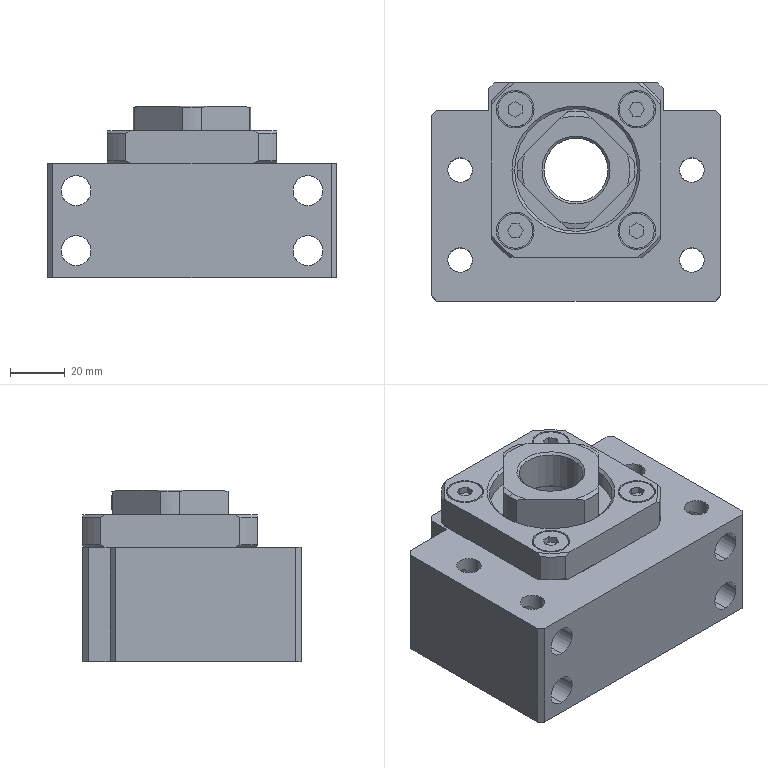Component | SolidWorks | BK_25-1 | 2 solids | 212 faces | volume 322317 mm3 | plane 93 | cylinder 89 | cone 28 | torus 2 | commonest cylinder face diameters 9 x24 12.8 x8 13.8 x8 11 x8 17.5 x8 43 x5 5 x4 45 x4